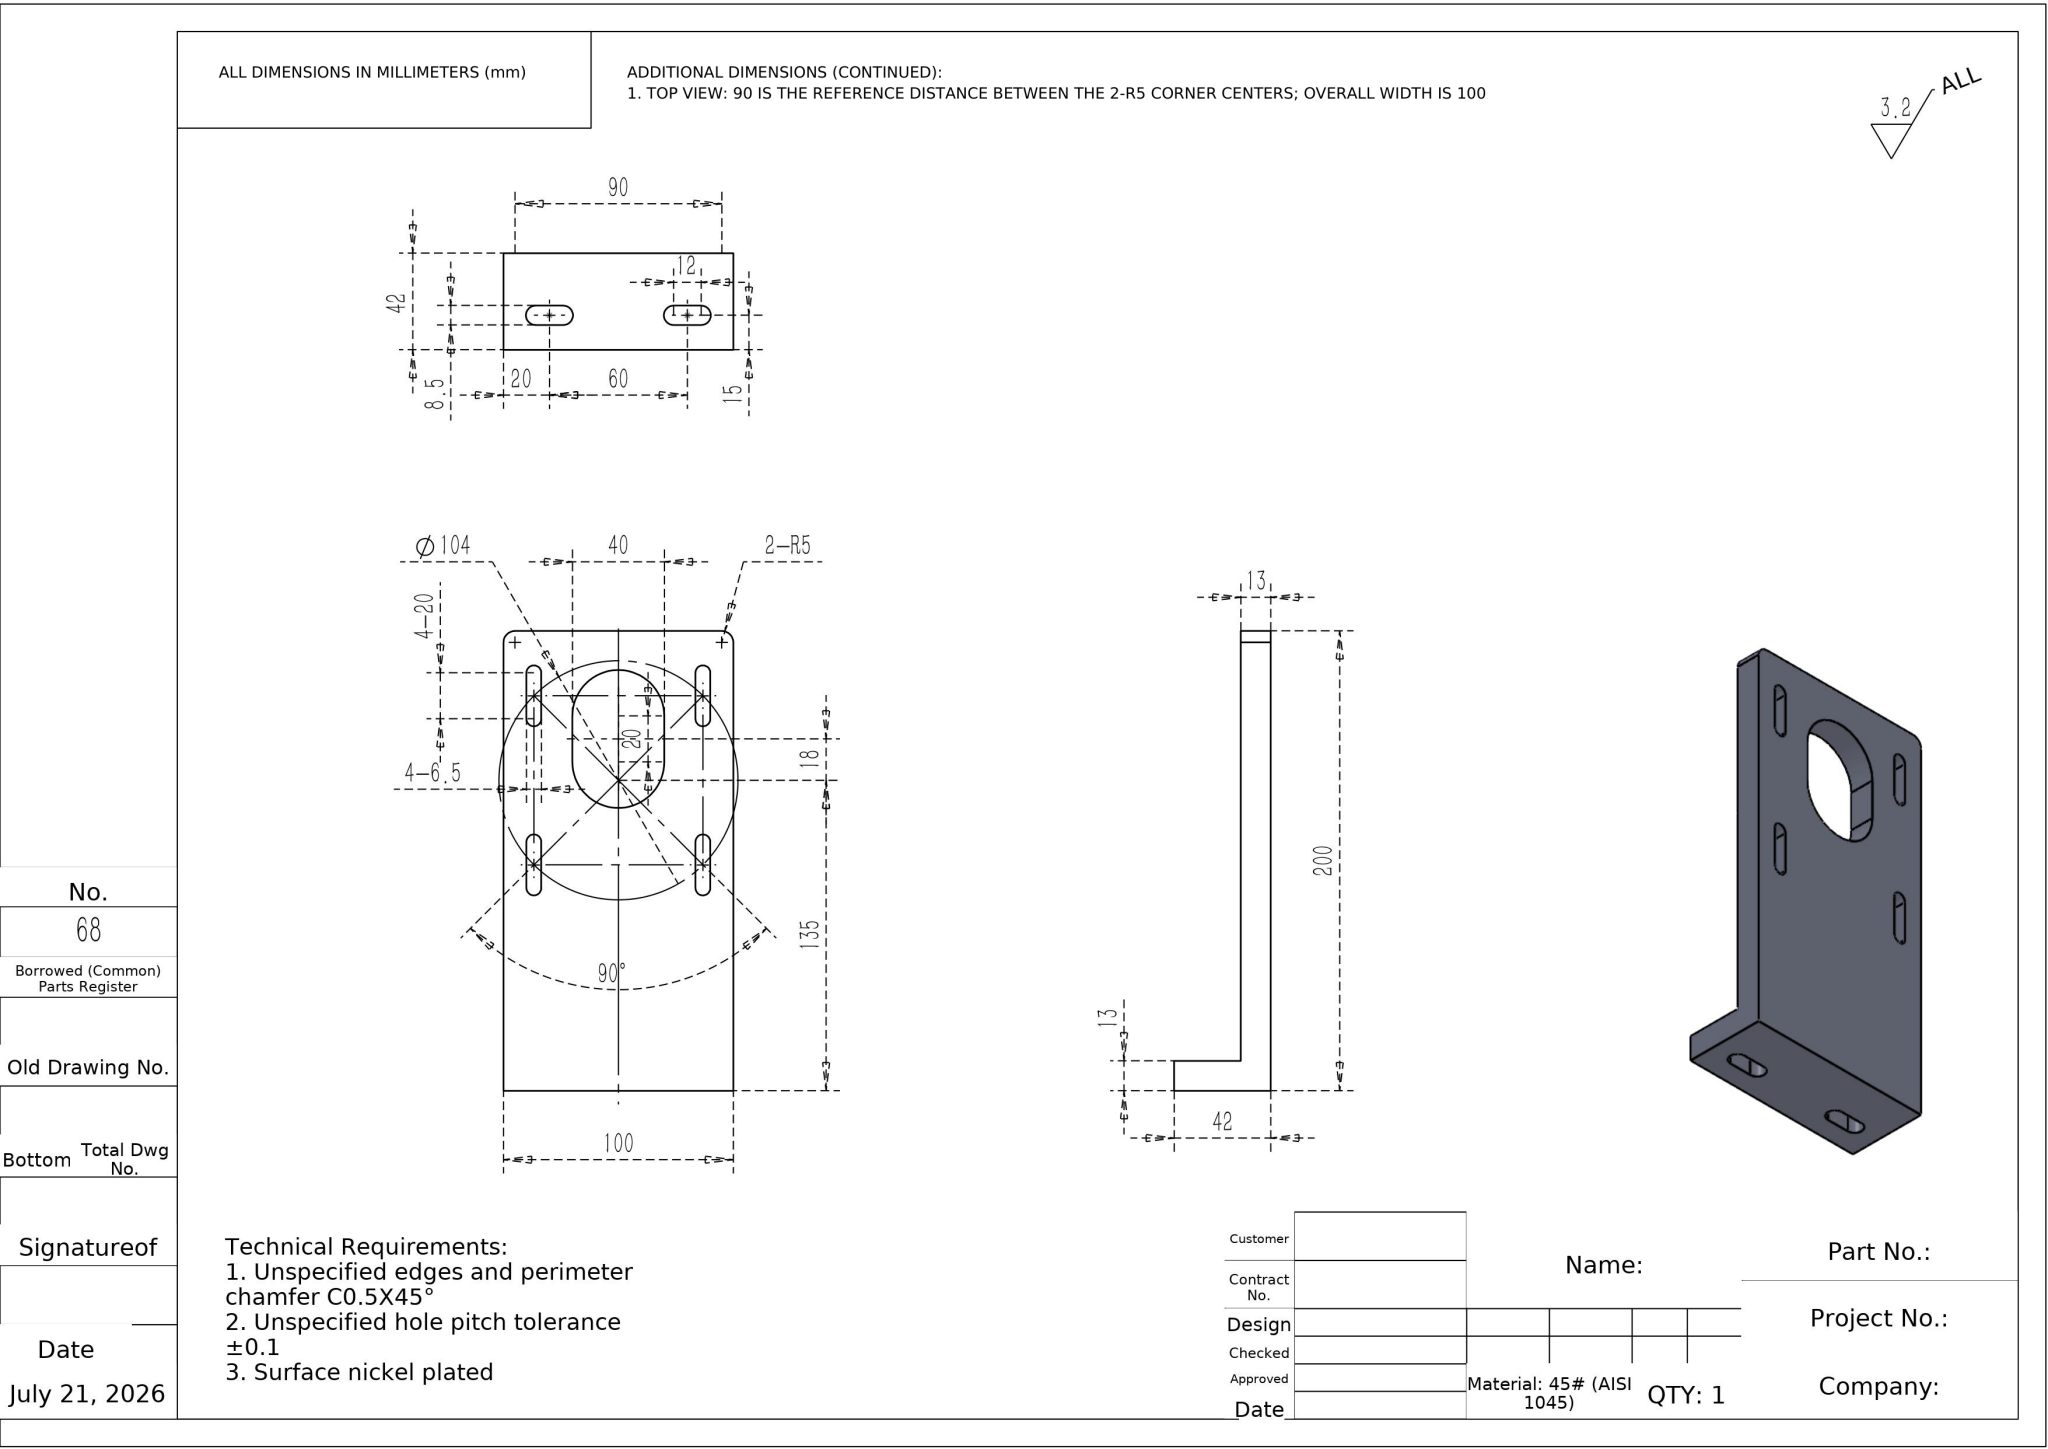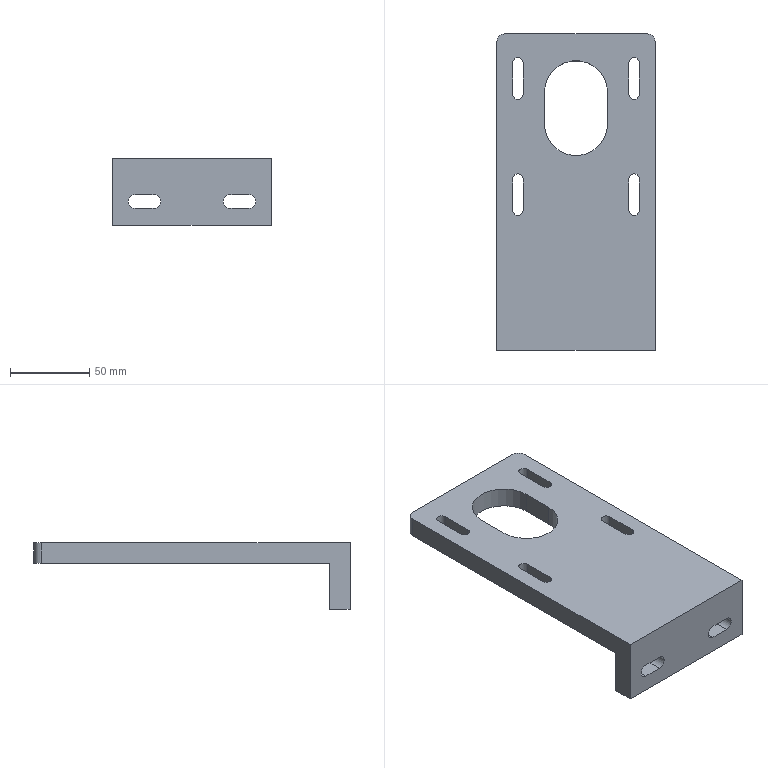Part | NX | mm | 1 solid | 38 faces | box 100 x 200 x 42 mm | volume 258211 mm3 | plane 22 | cylinder 16 | commonest cylinder face diameters 6.5 x8 8.5 x4 10 x2 40 x2